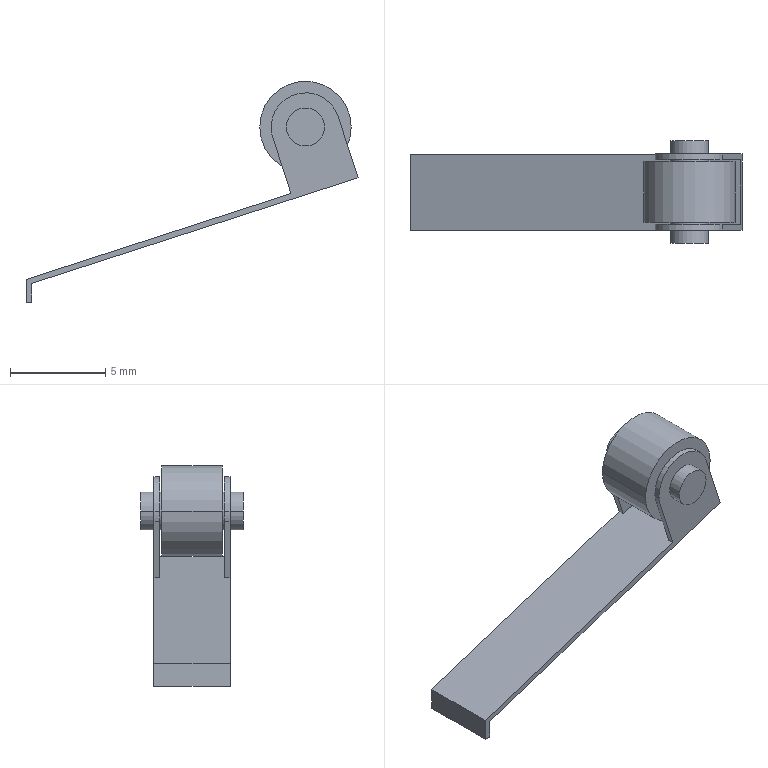Component | SolidWorks | SS_10GL2-1_SS_10GL2_ACTUATOR-1 | 1 solid | 30 faces | box 17.42 x 5.4 x 11.6 mm | volume 96 mm3 | plane 16 | cylinder 14 | commonest cylinder face diameters 2 x8 3.6 x4 4.8 x2
STEP:
#1=COLOUR_RGB('',0.7922,0.8196,0.9333);
#2=FILL_AREA_STYLE_COLOUR('',#1);
#3=FILL_AREA_STYLE('',(#2));
#4=SURFACE_STYLE_FILL_AREA(#3);
#5=SURFACE_SIDE_STYLE('',(#4));
#6=SURFACE_STYLE_USAGE(.BOTH.,#5);
#7=PRESENTATION_STYLE_ASSIGNMENT((#6));
#8=CARTESIAN_POINT('',(11.66,-32.095,0.3882));
#9=VERTEX_POINT('',#8);
#10=CARTESIAN_POINT('',(11.581,-32.095,0.3882));
#11=VERTEX_POINT('',#10);
#12=CARTESIAN_POINT('',(11.621,-32.095,0.3882));
#13=DIRECTION('',(0.,-1.,-0.));
#14=DIRECTION('',(1.,0.,0.));
#15=AXIS2_PLACEMENT_3D('',#12,#13,#14);
#16=CIRCLE('',#15,0.03937);
#17=EDGE_CURVE('',#9,#11,#16,.T.);
#18=ORIENTED_EDGE('',*,*,#17,.T.);
#19=CARTESIAN_POINT('',(11.581,-32.122,0.3882));
#20=VERTEX_POINT('',#19);
#21=CARTESIAN_POINT('',(11.581,-32.095,0.3882));
#22=DIRECTION('',(0.,-1.,-0.));
#23=VECTOR('',#22,39.37);
#24=LINE('',#21,#23);
#25=EDGE_CURVE('',#11,#20,#24,.T.);
#26=ORIENTED_EDGE('',*,*,#25,.T.);
#27=CARTESIAN_POINT('',(11.66,-32.122,0.3882));
#28=VERTEX_POINT('',#27);
#29=CARTESIAN_POINT('',(11.621,-32.122,0.3882));
#30=DIRECTION('',(0.,-1.,-0.));
#31=DIRECTION('',(1.,0.,0.));
#32=AXIS2_PLACEMENT_3D('',#29,#30,#31);
#33=CIRCLE('',#32,0.03937);
#34=EDGE_CURVE('',#28,#20,#33,.T.);
#35=ORIENTED_EDGE('',*,*,#34,.F.);
#36=CARTESIAN_POINT('',(11.66,-32.095,0.3882));
#37=DIRECTION('',(0.,-1.,-0.));
#38=VECTOR('',#37,39.37);
#39=LINE('',#36,#38);
#40=EDGE_CURVE('',#9,#28,#39,.T.);
#41=ORIENTED_EDGE('',*,*,#40,.F.);
#42=EDGE_LOOP('',(#18,#26,#35,#41));
#43=FACE_OUTER_BOUND('',#42,.T.);
#44=CARTESIAN_POINT('',(11.621,-32.095,0.3882));
#45=DIRECTION('',(0.,-1.,-0.));
#46=DIRECTION('',(1.,0.,0.));
#47=AXIS2_PLACEMENT_3D('',#44,#45,#46);
#48=CYLINDRICAL_SURFACE('',#47,0.03937);
#49=ADVANCED_FACE('',(#43),#48,.T.);
#50=CARTESIAN_POINT('',(11.553,-32.134,0.3664));
#51=VERTEX_POINT('',#50);
#52=CARTESIAN_POINT('',(11.55,-32.134,0.3882));
#53=VERTEX_POINT('',#52);
#54=CARTESIAN_POINT('',(11.621,-32.134,0.3882));
#55=DIRECTION('',(-0.,1.,0.));
#56=DIRECTION('',(-1.,0.,-0.));
#57=AXIS2_PLACEMENT_3D('',#54,#55,#56);
#58=CIRCLE('',#57,0.07087);
#59=EDGE_CURVE('',#51,#53,#58,.T.);
#60=ORIENTED_EDGE('',*,*,#59,.T.);
#61=CARTESIAN_POINT('',(11.55,-32.122,0.3882));
#62=VERTEX_POINT('',#61);
#63=CARTESIAN_POINT('',(11.55,-32.28,0.3882));
#64=DIRECTION('',(-0.,1.,0.));
#65=VECTOR('',#64,39.37);
#66=LINE('',#63,#65);
#67=EDGE_CURVE('',#53,#62,#66,.T.);
#68=ORIENTED_EDGE('',*,*,#67,.T.);
#69=CARTESIAN_POINT('',(11.553,-32.122,0.3664));
#70=VERTEX_POINT('',#69);
#71=CARTESIAN_POINT('',(11.621,-32.122,0.3882));
#72=DIRECTION('',(-0.,1.,0.));
#73=DIRECTION('',(-1.,0.,-0.));
#74=AXIS2_PLACEMENT_3D('',#71,#72,#73);
#75=CIRCLE('',#74,0.07087);
#76=EDGE_CURVE('',#70,#62,#75,.T.);
#77=ORIENTED_EDGE('',*,*,#76,.F.);
#78=CARTESIAN_POINT('',(11.553,-32.28,0.3664));
#79=DIRECTION('',(0.,-1.,-0.));
#80=VECTOR('',#79,39.37);
#81=LINE('',#78,#80);
#82=EDGE_CURVE('',#70,#51,#81,.T.);
#83=ORIENTED_EDGE('',*,*,#82,.T.);
#84=EDGE_LOOP('',(#60,#68,#77,#83));
#85=FACE_OUTER_BOUND('',#84,.T.);
#86=CARTESIAN_POINT('',(11.621,-32.28,0.3882));
#87=DIRECTION('',(-0.,1.,0.));
#88=DIRECTION('',(-1.,0.,-0.));
#89=AXIS2_PLACEMENT_3D('',#86,#87,#88);
#90=CYLINDRICAL_SURFACE('',#89,0.07087);
#91=ADVANCED_FACE('',(#85),#90,.T.);
#92=CARTESIAN_POINT('',(11.581,-32.307,0.3882));
#93=VERTEX_POINT('',#92);
#94=CARTESIAN_POINT('',(11.66,-32.307,0.3882));
#95=VERTEX_POINT('',#94);
#96=CARTESIAN_POINT('',(11.621,-32.307,0.3882));
#97=DIRECTION('',(-0.,1.,0.));
#98=DIRECTION('',(-1.,0.,-0.));
#99=AXIS2_PLACEMENT_3D('',#96,#97,#98);
#100=CIRCLE('',#99,0.03937);
#101=EDGE_CURVE('',#93,#95,#100,.T.);
#102=ORIENTED_EDGE('',*,*,#101,.T.);
#103=CARTESIAN_POINT('',(11.66,-32.28,0.3882));
#104=VERTEX_POINT('',#103);
#105=CARTESIAN_POINT('',(11.66,-32.307,0.3882));
#106=DIRECTION('',(-0.,1.,0.));
#107=VECTOR('',#106,39.37);
#108=LINE('',#105,#107);
#109=EDGE_CURVE('',#95,#104,#108,.T.);
#110=ORIENTED_EDGE('',*,*,#109,.T.);
#111=CARTESIAN_POINT('',(11.581,-32.28,0.3882));
#112=VERTEX_POINT('',#111);
#113=CARTESIAN_POINT('',(11.621,-32.28,0.3882));
#114=DIRECTION('',(0.,-1.,-0.));
#115=DIRECTION('',(-1.,0.,-0.));
#116=AXIS2_PLACEMENT_3D('',#113,#114,#115);
#117=CIRCLE('',#116,0.03937);
#118=EDGE_CURVE('',#104,#112,#117,.T.);
#119=ORIENTED_EDGE('',*,*,#118,.T.);
#120=CARTESIAN_POINT('',(11.581,-32.307,0.3882));
#121=DIRECTION('',(-0.,1.,0.));
#122=VECTOR('',#121,39.37);
#123=LINE('',#120,#122);
#124=EDGE_CURVE('',#93,#112,#123,.T.);
#125=ORIENTED_EDGE('',*,*,#124,.F.);
#126=EDGE_LOOP('',(#102,#110,#119,#125));
#127=FACE_OUTER_BOUND('',#126,.T.);
#128=CARTESIAN_POINT('',(11.621,-32.307,0.3882));
#129=DIRECTION('',(-0.,1.,0.));
#130=DIRECTION('',(-1.,0.,-0.));
#131=AXIS2_PLACEMENT_3D('',#128,#129,#130);
#132=CYLINDRICAL_SURFACE('',#131,0.03937);
#133=ADVANCED_FACE('',(#127),#132,.T.);
#134=CARTESIAN_POINT('',(11.553,-32.28,0.3664));
#135=VERTEX_POINT('',#134);
#136=CARTESIAN_POINT('',(11.55,-32.28,0.3882));
#137=VERTEX_POINT('',#136);
#138=CARTESIAN_POINT('',(11.621,-32.28,0.3882));
#139=DIRECTION('',(-0.,1.,0.));
#140=DIRECTION('',(-1.,0.,-0.));
#141=AXIS2_PLACEMENT_3D('',#138,#139,#140);
#142=CIRCLE('',#141,0.07087);
#143=EDGE_CURVE('',#135,#137,#142,.T.);
#144=ORIENTED_EDGE('',*,*,#143,.T.);
#145=CARTESIAN_POINT('',(11.55,-32.268,0.3882));
#146=VERTEX_POINT('',#145);
#147=CARTESIAN_POINT('',(11.55,-32.28,0.3882));
#148=DIRECTION('',(-0.,1.,0.));
#149=VECTOR('',#148,39.37);
#150=LINE('',#147,#149);
#151=EDGE_CURVE('',#137,#146,#150,.T.);
#152=ORIENTED_EDGE('',*,*,#151,.T.);
#153=CARTESIAN_POINT('',(11.553,-32.268,0.3664));
#154=VERTEX_POINT('',#153);
#155=CARTESIAN_POINT('',(11.621,-32.268,0.3882));
#156=DIRECTION('',(-0.,1.,0.));
#157=DIRECTION('',(-1.,0.,-0.));
#158=AXIS2_PLACEMENT_3D('',#155,#156,#157);
#159=CIRCLE('',#158,0.07087);
#160=EDGE_CURVE('',#154,#146,#159,.T.);
#161=ORIENTED_EDGE('',*,*,#160,.F.);
#162=CARTESIAN_POINT('',(11.553,-32.28,0.3664));
#163=DIRECTION('',(0.,-1.,-0.));
#164=VECTOR('',#163,39.37);
#165=LINE('',#162,#164);
#166=EDGE_CURVE('',#154,#135,#165,.T.);
#167=ORIENTED_EDGE('',*,*,#166,.T.);
#168=EDGE_LOOP('',(#144,#152,#161,#167));
#169=FACE_OUTER_BOUND('',#168,.T.);
#170=CARTESIAN_POINT('',(11.621,-32.28,0.3882));
#171=DIRECTION('',(-0.,1.,0.));
#172=DIRECTION('',(-1.,0.,-0.));
#173=AXIS2_PLACEMENT_3D('',#170,#171,#172);
#174=CYLINDRICAL_SURFACE('',#173,0.07087);
#175=ADVANCED_FACE('',(#169),#174,.T.);
#176=CARTESIAN_POINT('',(11.66,-32.268,0.3882));
#177=VERTEX_POINT('',#176);
#178=CARTESIAN_POINT('',(11.581,-32.268,0.3882));
#179=VERTEX_POINT('',#178);
#180=CARTESIAN_POINT('',(11.621,-32.268,0.3882));
#181=DIRECTION('',(0.,-1.,-0.));
#182=DIRECTION('',(-1.,0.,-0.));
#183=AXIS2_PLACEMENT_3D('',#180,#181,#182);
#184=CIRCLE('',#183,0.03937);
#185=EDGE_CURVE('',#177,#179,#184,.T.);
#186=ORIENTED_EDGE('',*,*,#185,.F.);
#187=CARTESIAN_POINT('',(11.66,-32.264,0.3882));
#188=VERTEX_POINT('',#187);
#189=CARTESIAN_POINT('',(11.66,-32.307,0.3882));
#190=DIRECTION('',(-0.,1.,0.));
#191=VECTOR('',#190,39.37);
#192=LINE('',#189,#191);
#193=EDGE_CURVE('',#177,#188,#192,.T.);
#194=ORIENTED_EDGE('',*,*,#193,.T.);
#195=CARTESIAN_POINT('',(11.581,-32.264,0.3882));
#196=VERTEX_POINT('',#195);
#197=CARTESIAN_POINT('',(11.621,-32.264,0.3882));
#198=DIRECTION('',(0.,-1.,-0.));
#199=DIRECTION('',(-1.,0.,-0.));
#200=AXIS2_PLACEMENT_3D('',#197,#198,#199);
#201=CIRCLE('',#200,0.03937);
#202=EDGE_CURVE('',#188,#196,#201,.T.);
#203=ORIENTED_EDGE('',*,*,#202,.T.);
#204=CARTESIAN_POINT('',(11.581,-32.307,0.3882));
#205=DIRECTION('',(-0.,1.,0.));
#206=VECTOR('',#205,39.37);
#207=LINE('',#204,#206);
#208=EDGE_CURVE('',#179,#196,#207,.T.);
#209=ORIENTED_EDGE('',*,*,#208,.F.);
#210=EDGE_LOOP('',(#186,#194,#203,#209));
#211=FACE_OUTER_BOUND('',#210,.T.);
#212=CARTESIAN_POINT('',(11.621,-32.307,0.3882));
#213=DIRECTION('',(-0.,1.,0.));
#214=DIRECTION('',(-1.,0.,-0.));
#215=AXIS2_PLACEMENT_3D('',#212,#213,#214);
#216=CYLINDRICAL_SURFACE('',#215,0.03937);
#217=ADVANCED_FACE('',(#211),#216,.T.);
#218=CARTESIAN_POINT('',(11.66,-32.134,0.3882));
#219=VERTEX_POINT('',#218);
#220=CARTESIAN_POINT('',(11.581,-32.134,0.3882));
#221=VERTEX_POINT('',#220);
#222=CARTESIAN_POINT('',(11.621,-32.134,0.3882));
#223=DIRECTION('',(0.,-1.,-0.));
#224=DIRECTION('',(1.,0.,0.));
#225=AXIS2_PLACEMENT_3D('',#222,#223,#224);
#226=CIRCLE('',#225,0.03937);
#227=EDGE_CURVE('',#219,#221,#226,.T.);
#228=ORIENTED_EDGE('',*,*,#227,.T.);
#229=CARTESIAN_POINT('',(11.581,-32.138,0.3882));
#230=VERTEX_POINT('',#229);
#231=CARTESIAN_POINT('',(11.581,-32.095,0.3882));
#232=DIRECTION('',(0.,-1.,-0.));
#233=VECTOR('',#232,39.37);
#234=LINE('',#231,#233);
#235=EDGE_CURVE('',#221,#230,#234,.T.);
#236=ORIENTED_EDGE('',*,*,#235,.T.);
#237=CARTESIAN_POINT('',(11.66,-32.138,0.3882));
#238=VERTEX_POINT('',#237);
#239=CARTESIAN_POINT('',(11.621,-32.138,0.3882));
#240=DIRECTION('',(-0.,1.,0.));
#241=DIRECTION('',(1.,0.,0.));
#242=AXIS2_PLACEMENT_3D('',#239,#240,#241);
#243=CIRCLE('',#242,0.03937);
#244=EDGE_CURVE('',#230,#238,#243,.T.);
#245=ORIENTED_EDGE('',*,*,#244,.T.);
#246=CARTESIAN_POINT('',(11.66,-32.095,0.3882));
#247=DIRECTION('',(0.,-1.,-0.));
#248=VECTOR('',#247,39.37);
#249=LINE('',#246,#248);
#250=EDGE_CURVE('',#219,#238,#249,.T.);
#251=ORIENTED_EDGE('',*,*,#250,.F.);
#252=EDGE_LOOP('',(#228,#236,#245,#251));
#253=FACE_OUTER_BOUND('',#252,.T.);
#254=CARTESIAN_POINT('',(11.621,-32.095,0.3882));
#255=DIRECTION('',(0.,-1.,-0.));
#256=DIRECTION('',(1.,0.,0.));
#257=AXIS2_PLACEMENT_3D('',#254,#255,#256);
#258=CYLINDRICAL_SURFACE('',#257,0.03937);
#259=ADVANCED_FACE('',(#253),#258,.T.);
#260=CARTESIAN_POINT('',(11.526,-32.138,0.3882));
#261=VERTEX_POINT('',#260);
#262=CARTESIAN_POINT('',(11.715,-32.138,0.3882));
#263=VERTEX_POINT('',#262);
#264=CARTESIAN_POINT('',(11.621,-32.138,0.3882));
#265=DIRECTION('',(-0.,1.,0.));
#266=DIRECTION('',(1.,0.,0.));
#267=AXIS2_PLACEMENT_3D('',#264,#265,#266);
#268=CIRCLE('',#267,0.09449);
#269=EDGE_CURVE('',#261,#263,#268,.T.);
#270=ORIENTED_EDGE('',*,*,#269,.F.);
#271=CARTESIAN_POINT('',(11.526,-32.264,0.3882));
#272=VERTEX_POINT('',#271);
#273=CARTESIAN_POINT('',(11.526,-32.138,0.3882));
#274=DIRECTION('',(0.,-1.,-0.));
#275=VECTOR('',#274,39.37);
#276=LINE('',#273,#275);
#277=EDGE_CURVE('',#261,#272,#276,.T.);
#278=ORIENTED_EDGE('',*,*,#277,.T.);
#279=CARTESIAN_POINT('',(11.715,-32.264,0.3882));
#280=VERTEX_POINT('',#279);
#281=CARTESIAN_POINT('',(11.621,-32.264,0.3882));
#282=DIRECTION('',(-0.,1.,0.));
#283=DIRECTION('',(1.,0.,0.));
#284=AXIS2_PLACEMENT_3D('',#281,#282,#283);
#285=CIRCLE('',#284,0.09449);
#286=EDGE_CURVE('',#272,#280,#285,.T.);
#287=ORIENTED_EDGE('',*,*,#286,.T.);
#288=CARTESIAN_POINT('',(11.715,-32.138,0.3882));
#289=DIRECTION('',(0.,-1.,-0.));
#290=VECTOR('',#289,39.37);
#291=LINE('',#288,#290);
#292=EDGE_CURVE('',#263,#280,#291,.T.);
#293=ORIENTED_EDGE('',*,*,#292,.F.);
#294=EDGE_LOOP('',(#270,#278,#287,#293));
#295=FACE_OUTER_BOUND('',#294,.T.);
#296=CARTESIAN_POINT('',(11.621,-32.138,0.3882));
#297=DIRECTION('',(0.,-1.,-0.));
#298=DIRECTION('',(1.,0.,0.));
#299=AXIS2_PLACEMENT_3D('',#296,#297,#298);
#300=CYLINDRICAL_SURFACE('',#299,0.09449);
#301=ADVANCED_FACE('',(#295),#300,.T.);
#302=CARTESIAN_POINT('',(11.729,-32.28,0.2829));
#303=VERTEX_POINT('',#302);
#304=CARTESIAN_POINT('',(11.729,-32.122,0.2829));
#305=VERTEX_POINT('',#304);
#306=CARTESIAN_POINT('',(11.729,-32.28,0.2829));
#307=DIRECTION('',(-0.,1.,0.));
#308=VECTOR('',#307,39.37);
#309=LINE('',#306,#308);
#310=EDGE_CURVE('',#303,#305,#309,.T.);
#311=ORIENTED_EDGE('',*,*,#310,.F.);
#312=CARTESIAN_POINT('',(11.055,-32.28,0.06494));
#313=VERTEX_POINT('',#312);
#314=CARTESIAN_POINT('',(11.055,-32.28,0.06494));
#315=DIRECTION('',(0.9515,0.,0.3077));
#316=VECTOR('',#315,39.37);
#317=LINE('',#314,#316);
#318=EDGE_CURVE('',#313,#303,#317,.T.);
#319=ORIENTED_EDGE('',*,*,#318,.F.);
#320=CARTESIAN_POINT('',(11.055,-32.122,0.06494));
#321=VERTEX_POINT('',#320);
#322=CARTESIAN_POINT('',(11.055,-32.28,0.06494));
#323=DIRECTION('',(0.,-1.,-0.));
#324=VECTOR('',#323,39.37);
#325=LINE('',#322,#324);
#326=EDGE_CURVE('',#321,#313,#325,.T.);
#327=ORIENTED_EDGE('',*,*,#326,.F.);
#328=CARTESIAN_POINT('',(11.055,-32.122,0.06494));
#329=DIRECTION('',(-0.9515,-0.,-0.3077));
#330=VECTOR('',#329,39.37);
#331=LINE('',#328,#330);
#332=EDGE_CURVE('',#305,#321,#331,.T.);
#333=ORIENTED_EDGE('',*,*,#332,.F.);
#334=EDGE_LOOP('',(#311,#319,#327,#333));
#335=FACE_OUTER_BOUND('',#334,.T.);
#336=CARTESIAN_POINT('',(11.055,-32.28,0.06494));
#337=DIRECTION('',(-0.3077,-0.,0.9515));
#338=DIRECTION('',(-0.9515,-0.,-0.3077));
#339=AXIS2_PLACEMENT_3D('',#336,#337,#338);
#340=PLANE('',#339);
#341=ADVANCED_FACE('',(#335),#340,.F.);
#342=ORIENTED_EDGE('',*,*,#34,.T.);
#343=CARTESIAN_POINT('',(11.621,-32.122,0.3882));
#344=DIRECTION('',(0.,-1.,-0.));
#345=DIRECTION('',(1.,0.,0.));
#346=AXIS2_PLACEMENT_3D('',#343,#344,#345);
#347=CIRCLE('',#346,0.03937);
#348=EDGE_CURVE('',#20,#28,#347,.T.);
#349=ORIENTED_EDGE('',*,*,#348,.T.);
#350=EDGE_LOOP('',(#342,#349));
#351=FACE_BOUND('',#350,.T.);
#352=CARTESIAN_POINT('',(11.688,-32.122,0.41));
#353=VERTEX_POINT('',#352);
#354=CARTESIAN_POINT('',(11.688,-32.122,0.41));
#355=DIRECTION('',(0.3077,0.,-0.9515));
#356=VECTOR('',#355,39.37);
#357=LINE('',#354,#356);
#358=EDGE_CURVE('',#353,#305,#357,.T.);
#359=ORIENTED_EDGE('',*,*,#358,.T.);
#360=ORIENTED_EDGE('',*,*,#332,.T.);
#361=CARTESIAN_POINT('',(11.055,-32.122,0.02597));
#362=VERTEX_POINT('',#361);
#363=CARTESIAN_POINT('',(11.055,-32.122,0.3882));
#364=DIRECTION('',(0.,0.,-1.));
#365=VECTOR('',#364,39.37);
#366=LINE('',#363,#365);
#367=EDGE_CURVE('',#321,#362,#366,.T.);
#368=ORIENTED_EDGE('',*,*,#367,.T.);
#369=CARTESIAN_POINT('',(11.043,-32.122,0.02597));
#370=VERTEX_POINT('',#369);
#371=CARTESIAN_POINT('',(11.055,-32.122,0.02597));
#372=DIRECTION('',(-1.,-0.,-0.));
#373=VECTOR('',#372,39.37);
#374=LINE('',#371,#373);
#375=EDGE_CURVE('',#362,#370,#374,.T.);
#376=ORIENTED_EDGE('',*,*,#375,.T.);
#377=CARTESIAN_POINT('',(11.043,-32.122,0.07354));
#378=VERTEX_POINT('',#377);
#379=CARTESIAN_POINT('',(11.043,-32.122,0.07354));
#380=DIRECTION('',(-0.,-0.,1.));
#381=VECTOR('',#380,39.37);
#382=LINE('',#379,#381);
#383=EDGE_CURVE('',#370,#378,#382,.T.);
#384=ORIENTED_EDGE('',*,*,#383,.T.);
#385=CARTESIAN_POINT('',(11.591,-32.122,0.2506));
#386=VERTEX_POINT('',#385);
#387=CARTESIAN_POINT('',(11.043,-32.122,0.07354));
#388=DIRECTION('',(0.9515,0.,0.3077));
#389=VECTOR('',#388,39.37);
#390=LINE('',#387,#389);
#391=EDGE_CURVE('',#378,#386,#390,.T.);
#392=ORIENTED_EDGE('',*,*,#391,.T.);
#393=CARTESIAN_POINT('',(11.591,-32.122,0.2506));
#394=DIRECTION('',(-0.3077,-0.,0.9515));
#395=VECTOR('',#394,39.37);
#396=LINE('',#393,#395);
#397=EDGE_CURVE('',#386,#70,#396,.T.);
#398=ORIENTED_EDGE('',*,*,#397,.T.);
#399=ORIENTED_EDGE('',*,*,#76,.T.);
#400=CARTESIAN_POINT('',(11.621,-32.122,0.3882));
#401=DIRECTION('',(-0.,1.,0.));
#402=DIRECTION('',(-1.,0.,-0.));
#403=AXIS2_PLACEMENT_3D('',#400,#401,#402);
#404=CIRCLE('',#403,0.07087);
#405=EDGE_CURVE('',#62,#353,#404,.T.);
#406=ORIENTED_EDGE('',*,*,#405,.T.);
#407=EDGE_LOOP('',(#359,#360,#368,#376,#384,#392,#398,#399,#406));
#408=FACE_OUTER_BOUND('',#407,.T.);
#409=CARTESIAN_POINT('',(11.621,-32.122,0.3882));
#410=DIRECTION('',(-0.,1.,0.));
#411=DIRECTION('',(-1.,-0.,-0.));
#412=AXIS2_PLACEMENT_3D('',#409,#410,#411);
#413=PLANE('',#412);
#414=ADVANCED_FACE('',(#351,#408),#413,.T.);
#415=CARTESIAN_POINT('',(11.688,-32.28,0.41));
#416=VERTEX_POINT('',#415);
#417=CARTESIAN_POINT('',(11.688,-32.268,0.41));
#418=VERTEX_POINT('',#417);
#419=CARTESIAN_POINT('',(11.688,-32.28,0.41));
#420=DIRECTION('',(-0.,1.,0.));
#421=VECTOR('',#420,39.37);
#422=LINE('',#419,#421);
#423=EDGE_CURVE('',#416,#418,#422,.T.);
#424=ORIENTED_EDGE('',*,*,#423,.F.);
#425=CARTESIAN_POINT('',(11.688,-32.28,0.41));
#426=DIRECTION('',(-0.3077,-0.,0.9515));
#427=VECTOR('',#426,39.37);
#428=LINE('',#425,#427);
#429=EDGE_CURVE('',#303,#416,#428,.T.);
#430=ORIENTED_EDGE('',*,*,#429,.F.);
#431=ORIENTED_EDGE('',*,*,#310,.T.);
#432=ORIENTED_EDGE('',*,*,#358,.F.);
#433=CARTESIAN_POINT('',(11.688,-32.134,0.41));
#434=VERTEX_POINT('',#433);
#435=CARTESIAN_POINT('',(11.688,-32.28,0.41));
#436=DIRECTION('',(-0.,1.,0.));
#437=VECTOR('',#436,39.37);
#438=LINE('',#435,#437);
#439=EDGE_CURVE('',#434,#353,#438,.T.);
#440=ORIENTED_EDGE('',*,*,#439,.F.);
#441=CARTESIAN_POINT('',(11.726,-32.134,0.2942));
#442=VERTEX_POINT('',#441);
#443=CARTESIAN_POINT('',(11.688,-32.134,0.41));
#444=DIRECTION('',(-0.3077,-0.,0.9515));
#445=VECTOR('',#444,39.37);
#446=LINE('',#443,#445);
#447=EDGE_CURVE('',#442,#434,#446,.T.);
#448=ORIENTED_EDGE('',*,*,#447,.F.);
#449=CARTESIAN_POINT('',(11.726,-32.268,0.2942));
#450=VERTEX_POINT('',#449);
#451=CARTESIAN_POINT('',(11.726,-32.28,0.2942));
#452=DIRECTION('',(-0.,1.,0.));
#453=VECTOR('',#452,39.37);
#454=LINE('',#451,#453);
#455=EDGE_CURVE('',#450,#442,#454,.T.);
#456=ORIENTED_EDGE('',*,*,#455,.F.);
#457=CARTESIAN_POINT('',(11.688,-32.268,0.41));
#458=DIRECTION('',(0.3077,0.,-0.9515));
#459=VECTOR('',#458,39.37);
#460=LINE('',#457,#459);
#461=EDGE_CURVE('',#418,#450,#460,.T.);
#462=ORIENTED_EDGE('',*,*,#461,.F.);
#463=EDGE_LOOP('',(#424,#430,#431,#432,#440,#448,#456,#462));
#464=FACE_OUTER_BOUND('',#463,.T.);
#465=CARTESIAN_POINT('',(11.688,-32.28,0.41));
#466=DIRECTION('',(-0.9515,-0.,-0.3077));
#467=DIRECTION('',(0.3077,0.,-0.9515));
#468=AXIS2_PLACEMENT_3D('',#465,#466,#467);
#469=PLANE('',#468);
#470=ADVANCED_FACE('',(#464),#469,.F.);
#471=CARTESIAN_POINT('',(11.621,-32.28,0.3882));
#472=DIRECTION('',(0.,-1.,-0.));
#473=DIRECTION('',(-1.,0.,-0.));
#474=AXIS2_PLACEMENT_3D('',#471,#472,#473);
#475=CIRCLE('',#474,0.03937);
#476=EDGE_CURVE('',#112,#104,#475,.T.);
#477=ORIENTED_EDGE('',*,*,#476,.F.);
#478=ORIENTED_EDGE('',*,*,#118,.F.);
#479=EDGE_LOOP('',(#477,#478));
#480=FACE_BOUND('',#479,.T.);
#481=ORIENTED_EDGE('',*,*,#318,.T.);
#482=ORIENTED_EDGE('',*,*,#429,.T.);
#483=CARTESIAN_POINT('',(11.621,-32.28,0.3882));
#484=DIRECTION('',(-0.,1.,0.));
#485=DIRECTION('',(-1.,0.,-0.));
#486=AXIS2_PLACEMENT_3D('',#483,#484,#485);
#487=CIRCLE('',#486,0.07087);
#488=EDGE_CURVE('',#137,#416,#487,.T.);
#489=ORIENTED_EDGE('',*,*,#488,.F.);
#490=ORIENTED_EDGE('',*,*,#143,.F.);
#491=CARTESIAN_POINT('',(11.591,-32.28,0.2506));
#492=VERTEX_POINT('',#491);
#493=CARTESIAN_POINT('',(11.591,-32.28,0.2506));
#494=DIRECTION('',(-0.3077,-0.,0.9515));
#495=VECTOR('',#494,39.37);
#496=LINE('',#493,#495);
#497=EDGE_CURVE('',#492,#135,#496,.T.);
#498=ORIENTED_EDGE('',*,*,#497,.F.);
#499=CARTESIAN_POINT('',(11.043,-32.28,0.07354));
#500=VERTEX_POINT('',#499);
#501=CARTESIAN_POINT('',(11.043,-32.28,0.07354));
#502=DIRECTION('',(0.9515,0.,0.3077));
#503=VECTOR('',#502,39.37);
#504=LINE('',#501,#503);
#505=EDGE_CURVE('',#500,#492,#504,.T.);
#506=ORIENTED_EDGE('',*,*,#505,.F.);
#507=CARTESIAN_POINT('',(11.043,-32.28,0.02597));
#508=VERTEX_POINT('',#507);
#509=CARTESIAN_POINT('',(11.043,-32.28,0.07354));
#510=DIRECTION('',(0.,0.,-1.));
#511=VECTOR('',#510,39.37);
#512=LINE('',#509,#511);
#513=EDGE_CURVE('',#500,#508,#512,.T.);
#514=ORIENTED_EDGE('',*,*,#513,.T.);
#515=CARTESIAN_POINT('',(11.055,-32.28,0.02597));
#516=VERTEX_POINT('',#515);
#517=CARTESIAN_POINT('',(11.055,-32.28,0.02597));
#518=DIRECTION('',(1.,0.,0.));
#519=VECTOR('',#518,39.37);
#520=LINE('',#517,#519);
#521=EDGE_CURVE('',#508,#516,#520,.T.);
#522=ORIENTED_EDGE('',*,*,#521,.T.);
#523=CARTESIAN_POINT('',(11.055,-32.28,0.3882));
#524=DIRECTION('',(0.,0.,-1.));
#525=VECTOR('',#524,39.37);
#526=LINE('',#523,#525);
#527=EDGE_CURVE('',#313,#516,#526,.T.);
#528=ORIENTED_EDGE('',*,*,#527,.F.);
#529=EDGE_LOOP('',(#481,#482,#489,#490,#498,#506,#514,#522,#528));
#530=FACE_OUTER_BOUND('',#529,.T.);
#531=CARTESIAN_POINT('',(11.621,-32.28,0.3882));
#532=DIRECTION('',(-0.,1.,0.));
#533=DIRECTION('',(-1.,-0.,-0.));
#534=AXIS2_PLACEMENT_3D('',#531,#532,#533);
#535=PLANE('',#534);
#536=ADVANCED_FACE('',(#480,#530),#535,.F.);
#537=ORIENTED_EDGE('',*,*,#326,.T.);
#538=ORIENTED_EDGE('',*,*,#527,.T.);
#539=CARTESIAN_POINT('',(11.055,-32.28,0.02597));
#540=DIRECTION('',(0.,-1.,-0.));
#541=VECTOR('',#540,39.37);
#542=LINE('',#539,#541);
#543=EDGE_CURVE('',#362,#516,#542,.T.);
#544=ORIENTED_EDGE('',*,*,#543,.F.);
#545=ORIENTED_EDGE('',*,*,#367,.F.);
#546=EDGE_LOOP('',(#537,#538,#544,#545));
#547=FACE_OUTER_BOUND('',#546,.T.);
#548=CARTESIAN_POINT('',(11.055,-32.28,0.02597));
#549=DIRECTION('',(-1.,-0.,-0.));
#550=DIRECTION('',(0.,-1.,-0.));
#551=AXIS2_PLACEMENT_3D('',#548,#549,#550);
#552=PLANE('',#551);
#553=ADVANCED_FACE('',(#547),#552,.F.);
#554=ORIENTED_EDGE('',*,*,#25,.F.);
#555=CARTESIAN_POINT('',(11.621,-32.095,0.3882));
#556=DIRECTION('',(0.,-1.,-0.));
#557=DIRECTION('',(1.,0.,0.));
#558=AXIS2_PLACEMENT_3D('',#555,#556,#557);
#559=CIRCLE('',#558,0.03937);
#560=EDGE_CURVE('',#11,#9,#559,.T.);
#561=ORIENTED_EDGE('',*,*,#560,.T.);
#562=ORIENTED_EDGE('',*,*,#40,.T.);
#563=ORIENTED_EDGE('',*,*,#348,.F.);
#564=EDGE_LOOP('',(#554,#561,#562,#563));
#565=FACE_OUTER_BOUND('',#564,.T.);
#566=CARTESIAN_POINT('',(11.621,-32.095,0.3882));
#567=DIRECTION('',(0.,-1.,-0.));
#568=DIRECTION('',(1.,0.,0.));
#569=AXIS2_PLACEMENT_3D('',#566,#567,#568);
#570=CYLINDRICAL_SURFACE('',#569,0.03937);
#571=ADVANCED_FACE('',(#565),#570,.T.);
#572=ORIENTED_EDGE('',*,*,#67,.F.);
#573=CARTESIAN_POINT('',(11.621,-32.134,0.3882));
#574=DIRECTION('',(-0.,1.,0.));
#575=DIRECTION('',(-1.,0.,-0.));
#576=AXIS2_PLACEMENT_3D('',#573,#574,#575);
#577=CIRCLE('',#576,0.07087);
#578=EDGE_CURVE('',#53,#434,#577,.T.);
#579=ORIENTED_EDGE('',*,*,#578,.T.);
#580=ORIENTED_EDGE('',*,*,#439,.T.);
#581=ORIENTED_EDGE('',*,*,#405,.F.);
#582=EDGE_LOOP('',(#572,#579,#580,#581));
#583=FACE_OUTER_BOUND('',#582,.T.);
#584=CARTESIAN_POINT('',(11.621,-32.28,0.3882));
#585=DIRECTION('',(-0.,1.,0.));
#586=DIRECTION('',(-1.,0.,-0.));
#587=AXIS2_PLACEMENT_3D('',#584,#585,#586);
#588=CYLINDRICAL_SURFACE('',#587,0.07087);
#589=ADVANCED_FACE('',(#583),#588,.T.);
#590=CARTESIAN_POINT('',(11.591,-32.134,0.2506));
#591=VERTEX_POINT('',#590);
#592=CARTESIAN_POINT('',(11.591,-32.134,0.2506));
#593=DIRECTION('',(0.3077,0.,-0.9515));
#594=VECTOR('',#593,39.37);
#595=LINE('',#592,#594);
#596=EDGE_CURVE('',#51,#591,#595,.T.);
#597=ORIENTED_EDGE('',*,*,#596,.F.);
#598=ORIENTED_EDGE('',*,*,#82,.F.);
#599=ORIENTED_EDGE('',*,*,#397,.F.);
#600=CARTESIAN_POINT('',(11.591,-32.28,0.2506));
#601=DIRECTION('',(-0.,1.,0.));
#602=VECTOR('',#601,39.37);
#603=LINE('',#600,#602);
#604=EDGE_CURVE('',#591,#386,#603,.T.);
#605=ORIENTED_EDGE('',*,*,#604,.F.);
#606=EDGE_LOOP('',(#597,#598,#599,#605));
#607=FACE_OUTER_BOUND('',#606,.T.);
#608=CARTESIAN_POINT('',(11.591,-32.28,0.2506));
#609=DIRECTION('',(0.9515,0.,0.3077));
#610=DIRECTION('',(-0.3077,-0.,0.9515));
#611=AXIS2_PLACEMENT_3D('',#608,#609,#610);
#612=PLANE('',#611);
#613=ADVANCED_FACE('',(#607),#612,.F.);
#614=CARTESIAN_POINT('',(11.043,-32.28,0.07354));
#615=DIRECTION('',(-0.,1.,0.));
#616=VECTOR('',#615,39.37);
#617=LINE('',#614,#616);
#618=EDGE_CURVE('',#500,#378,#617,.T.);
#619=ORIENTED_EDGE('',*,*,#618,.F.);
#620=ORIENTED_EDGE('',*,*,#505,.T.);
#621=CARTESIAN_POINT('',(11.591,-32.268,0.2506));
#622=VERTEX_POINT('',#621);
#623=CARTESIAN_POINT('',(11.591,-32.28,0.2506));
#624=DIRECTION('',(0.,-1.,-0.));
#625=VECTOR('',#624,39.37);
#626=LINE('',#623,#625);
#627=EDGE_CURVE('',#622,#492,#626,.T.);
#628=ORIENTED_EDGE('',*,*,#627,.F.);
#629=CARTESIAN_POINT('',(11.591,-32.268,0.2506));
#630=DIRECTION('',(-0.9515,-0.,-0.3077));
#631=VECTOR('',#630,39.37);
#632=LINE('',#629,#631);
#633=EDGE_CURVE('',#450,#622,#632,.T.);
#634=ORIENTED_EDGE('',*,*,#633,.F.);
#635=ORIENTED_EDGE('',*,*,#455,.T.);
#636=CARTESIAN_POINT('',(11.591,-32.134,0.2506));
#637=DIRECTION('',(0.9515,0.,0.3077));
#638=VECTOR('',#637,39.37);
#639=LINE('',#636,#638);
#640=EDGE_CURVE('',#591,#442,#639,.T.);
#641=ORIENTED_EDGE('',*,*,#640,.F.);
#642=ORIENTED_EDGE('',*,*,#604,.T.);
#643=ORIENTED_EDGE('',*,*,#391,.F.);
#644=EDGE_LOOP('',(#619,#620,#628,#634,#635,#641,#642,#643));
#645=FACE_OUTER_BOUND('',#644,.T.);
#646=CARTESIAN_POINT('',(11.591,-32.28,0.2506));
#647=DIRECTION('',(0.3077,0.,-0.9515));
#648=DIRECTION('',(0.9515,0.,0.3077));
#649=AXIS2_PLACEMENT_3D('',#646,#647,#648);
#650=PLANE('',#649);
#651=ADVANCED_FACE('',(#645),#650,.F.);
#652=CARTESIAN_POINT('',(11.621,-32.268,0.3882));
#653=DIRECTION('',(0.,-1.,-0.));
#654=DIRECTION('',(-1.,0.,-0.));
#655=AXIS2_PLACEMENT_3D('',#652,#653,#654);
#656=CIRCLE('',#655,0.03937);
#657=EDGE_CURVE('',#179,#177,#656,.T.);
#658=ORIENTED_EDGE('',*,*,#657,.T.);
#659=ORIENTED_EDGE('',*,*,#185,.T.);
#660=EDGE_LOOP('',(#658,#659));
#661=FACE_BOUND('',#660,.T.);
#662=ORIENTED_EDGE('',*,*,#160,.T.);
#663=CARTESIAN_POINT('',(11.621,-32.268,0.3882));
#664=DIRECTION('',(-0.,1.,0.));
#665=DIRECTION('',(-1.,0.,-0.));
#666=AXIS2_PLACEMENT_3D('',#663,#664,#665);
#667=CIRCLE('',#666,0.07087);
#668=EDGE_CURVE('',#146,#418,#667,.T.);
#669=ORIENTED_EDGE('',*,*,#668,.T.);
#670=ORIENTED_EDGE('',*,*,#461,.T.);
#671=ORIENTED_EDGE('',*,*,#633,.T.);
#672=CARTESIAN_POINT('',(11.591,-32.268,0.2506));
#673=DIRECTION('',(-0.3077,-0.,0.9515));
#674=VECTOR('',#673,39.37);
#675=LINE('',#672,#674);
#676=EDGE_CURVE('',#622,#154,#675,.T.);
#677=ORIENTED_EDGE('',*,*,#676,.T.);
#678=EDGE_LOOP('',(#662,#669,#670,#671,#677));
#679=FACE_OUTER_BOUND('',#678,.T.);
#680=CARTESIAN_POINT('',(11.621,-32.268,0.3882));
#681=DIRECTION('',(-0.,1.,0.));
#682=DIRECTION('',(-1.,-0.,-0.));
#683=AXIS2_PLACEMENT_3D('',#680,#681,#682);
#684=PLANE('',#683);
#685=ADVANCED_FACE('',(#661,#679),#684,.T.);
#686=ORIENTED_EDGE('',*,*,#227,.F.);
#687=CARTESIAN_POINT('',(11.621,-32.134,0.3882));
#688=DIRECTION('',(0.,-1.,-0.));
#689=DIRECTION('',(1.,0.,0.));
#690=AXIS2_PLACEMENT_3D('',#687,#688,#689);
#691=CIRCLE('',#690,0.03937);
#692=EDGE_CURVE('',#221,#219,#691,.T.);
#693=ORIENTED_EDGE('',*,*,#692,.F.);
#694=EDGE_LOOP('',(#686,#693));
#695=FACE_BOUND('',#694,.T.);
#696=ORIENTED_EDGE('',*,*,#640,.T.);
#697=ORIENTED_EDGE('',*,*,#447,.T.);
#698=ORIENTED_EDGE('',*,*,#578,.F.);
#699=ORIENTED_EDGE('',*,*,#59,.F.);
#700=ORIENTED_EDGE('',*,*,#596,.T.);
#701=EDGE_LOOP('',(#696,#697,#698,#699,#700));
#702=FACE_OUTER_BOUND('',#701,.T.);
#703=CARTESIAN_POINT('',(11.621,-32.134,0.3882));
#704=DIRECTION('',(-0.,1.,0.));
#705=DIRECTION('',(-1.,-0.,-0.));
#706=AXIS2_PLACEMENT_3D('',#703,#704,#705);
#707=PLANE('',#706);
#708=ADVANCED_FACE('',(#695,#702),#707,.F.);
#709=ORIENTED_EDGE('',*,*,#109,.F.);
#710=CARTESIAN_POINT('',(11.621,-32.307,0.3882));
#711=DIRECTION('',(-0.,1.,0.));
#712=DIRECTION('',(-1.,0.,-0.));
#713=AXIS2_PLACEMENT_3D('',#710,#711,#712);
#714=CIRCLE('',#713,0.03937);
#715=EDGE_CURVE('',#95,#93,#714,.T.);
#716=ORIENTED_EDGE('',*,*,#715,.T.);
#717=ORIENTED_EDGE('',*,*,#124,.T.);
#718=ORIENTED_EDGE('',*,*,#476,.T.);
#719=EDGE_LOOP('',(#709,#716,#717,#718));
#720=FACE_OUTER_BOUND('',#719,.T.);
#721=CARTESIAN_POINT('',(11.621,-32.307,0.3882));
#722=DIRECTION('',(-0.,1.,0.));
#723=DIRECTION('',(-1.,0.,-0.));
#724=AXIS2_PLACEMENT_3D('',#721,#722,#723);
#725=CYLINDRICAL_SURFACE('',#724,0.03937);
#726=ADVANCED_FACE('',(#720),#725,.T.);
#727=ORIENTED_EDGE('',*,*,#151,.F.);
#728=ORIENTED_EDGE('',*,*,#488,.T.);
#729=ORIENTED_EDGE('',*,*,#423,.T.);
#730=ORIENTED_EDGE('',*,*,#668,.F.);
#731=EDGE_LOOP('',(#727,#728,#729,#730));
#732=FACE_OUTER_BOUND('',#731,.T.);
#733=CARTESIAN_POINT('',(11.621,-32.28,0.3882));
#734=DIRECTION('',(-0.,1.,0.));
#735=DIRECTION('',(-1.,0.,-0.));
#736=AXIS2_PLACEMENT_3D('',#733,#734,#735);
#737=CYLINDRICAL_SURFACE('',#736,0.07087);
#738=ADVANCED_FACE('',(#732),#737,.T.);
#739=ORIENTED_EDGE('',*,*,#627,.T.);
#740=ORIENTED_EDGE('',*,*,#497,.T.);
#741=ORIENTED_EDGE('',*,*,#166,.F.);
#742=ORIENTED_EDGE('',*,*,#676,.F.);
#743=EDGE_LOOP('',(#739,#740,#741,#742));
#744=FACE_OUTER_BOUND('',#743,.T.);
#745=CARTESIAN_POINT('',(11.591,-32.28,0.2506));
#746=DIRECTION('',(0.9515,0.,0.3077));
#747=DIRECTION('',(-0.3077,-0.,0.9515));
#748=AXIS2_PLACEMENT_3D('',#745,#746,#747);
#749=PLANE('',#748);
#750=ADVANCED_FACE('',(#744),#749,.F.);
#751=ORIENTED_EDGE('',*,*,#543,.T.);
#752=ORIENTED_EDGE('',*,*,#521,.F.);
#753=CARTESIAN_POINT('',(11.043,-32.28,0.02597));
#754=DIRECTION('',(0.,-1.,-0.));
#755=VECTOR('',#754,39.37);
#756=LINE('',#753,#755);
#757=EDGE_CURVE('',#370,#508,#756,.T.);
#758=ORIENTED_EDGE('',*,*,#757,.F.);
#759=ORIENTED_EDGE('',*,*,#375,.F.);
#760=EDGE_LOOP('',(#751,#752,#758,#759));
#761=FACE_OUTER_BOUND('',#760,.T.);
#762=CARTESIAN_POINT('',(11.055,-32.28,0.02597));
#763=DIRECTION('',(-0.,-0.,1.));
#764=DIRECTION('',(0.,-1.,-0.));
#765=AXIS2_PLACEMENT_3D('',#762,#763,#764);
#766=PLANE('',#765);
#767=ADVANCED_FACE('',(#761),#766,.F.);
#768=ORIENTED_EDGE('',*,*,#17,.F.);
#769=ORIENTED_EDGE('',*,*,#560,.F.);
#770=EDGE_LOOP('',(#768,#769));
#771=FACE_OUTER_BOUND('',#770,.T.);
#772=CARTESIAN_POINT('',(11.621,-32.095,0.3882));
#773=DIRECTION('',(-0.,1.,0.));
#774=DIRECTION('',(-1.,-0.,-0.));
#775=AXIS2_PLACEMENT_3D('',#772,#773,#774);
#776=PLANE('',#775);
#777=ADVANCED_FACE('',(#771),#776,.T.);
#778=ORIENTED_EDGE('',*,*,#757,.T.);
#779=ORIENTED_EDGE('',*,*,#513,.F.);
#780=ORIENTED_EDGE('',*,*,#618,.T.);
#781=ORIENTED_EDGE('',*,*,#383,.F.);
#782=EDGE_LOOP('',(#778,#779,#780,#781));
#783=FACE_OUTER_BOUND('',#782,.T.);
#784=CARTESIAN_POINT('',(11.043,-32.28,0.07354));
#785=DIRECTION('',(1.,0.,0.));
#786=DIRECTION('',(-0.,-0.,1.));
#787=AXIS2_PLACEMENT_3D('',#784,#785,#786);
#788=PLANE('',#787);
#789=ADVANCED_FACE('',(#783),#788,.F.);
#790=ORIENTED_EDGE('',*,*,#193,.F.);
#791=ORIENTED_EDGE('',*,*,#657,.F.);
#792=ORIENTED_EDGE('',*,*,#208,.T.);
#793=CARTESIAN_POINT('',(11.621,-32.264,0.3882));
#794=DIRECTION('',(0.,-1.,-0.));
#795=DIRECTION('',(-1.,0.,-0.));
#796=AXIS2_PLACEMENT_3D('',#793,#794,#795);
#797=CIRCLE('',#796,0.03937);
#798=EDGE_CURVE('',#196,#188,#797,.T.);
#799=ORIENTED_EDGE('',*,*,#798,.T.);
#800=EDGE_LOOP('',(#790,#791,#792,#799));
#801=FACE_OUTER_BOUND('',#800,.T.);
#802=CARTESIAN_POINT('',(11.621,-32.307,0.3882));
#803=DIRECTION('',(-0.,1.,0.));
#804=DIRECTION('',(-1.,0.,-0.));
#805=AXIS2_PLACEMENT_3D('',#802,#803,#804);
#806=CYLINDRICAL_SURFACE('',#805,0.03937);
#807=ADVANCED_FACE('',(#801),#806,.T.);
#808=ORIENTED_EDGE('',*,*,#235,.F.);
#809=ORIENTED_EDGE('',*,*,#692,.T.);
#810=ORIENTED_EDGE('',*,*,#250,.T.);
#811=CARTESIAN_POINT('',(11.621,-32.138,0.3882));
#812=DIRECTION('',(-0.,1.,0.));
#813=DIRECTION('',(1.,0.,0.));
#814=AXIS2_PLACEMENT_3D('',#811,#812,#813);
#815=CIRCLE('',#814,0.03937);
#816=EDGE_CURVE('',#238,#230,#815,.T.);
#817=ORIENTED_EDGE('',*,*,#816,.T.);
#818=EDGE_LOOP('',(#808,#809,#810,#817));
#819=FACE_OUTER_BOUND('',#818,.T.);
#820=CARTESIAN_POINT('',(11.621,-32.095,0.3882));
#821=DIRECTION('',(0.,-1.,-0.));
#822=DIRECTION('',(1.,0.,0.));
#823=AXIS2_PLACEMENT_3D('',#820,#821,#822);
#824=CYLINDRICAL_SURFACE('',#823,0.03937);
#825=ADVANCED_FACE('',(#819),#824,.T.);
#826=ORIENTED_EDGE('',*,*,#101,.F.);
#827=ORIENTED_EDGE('',*,*,#715,.F.);
#828=EDGE_LOOP('',(#826,#827));
#829=FACE_OUTER_BOUND('',#828,.T.);
#830=CARTESIAN_POINT('',(11.621,-32.307,0.3882));
#831=DIRECTION('',(0.,-1.,-0.));
#832=DIRECTION('',(1.,0.,0.));
#833=AXIS2_PLACEMENT_3D('',#830,#831,#832);
#834=PLANE('',#833);
#835=ADVANCED_FACE('',(#829),#834,.T.);
#836=ORIENTED_EDGE('',*,*,#798,.F.);
#837=ORIENTED_EDGE('',*,*,#202,.F.);
#838=EDGE_LOOP('',(#836,#837));
#839=FACE_BOUND('',#838,.T.);
#840=CARTESIAN_POINT('',(11.621,-32.264,0.3882));
#841=DIRECTION('',(-0.,1.,0.));
#842=DIRECTION('',(1.,0.,0.));
#843=AXIS2_PLACEMENT_3D('',#840,#841,#842);
#844=CIRCLE('',#843,0.09449);
#845=EDGE_CURVE('',#280,#272,#844,.T.);
#846=ORIENTED_EDGE('',*,*,#845,.F.);
#847=ORIENTED_EDGE('',*,*,#286,.F.);
#848=EDGE_LOOP('',(#846,#847));
#849=FACE_OUTER_BOUND('',#848,.T.);
#850=CARTESIAN_POINT('',(11.621,-32.264,0.3882));
#851=DIRECTION('',(-0.,1.,0.));
#852=DIRECTION('',(-1.,-0.,-0.));
#853=AXIS2_PLACEMENT_3D('',#850,#851,#852);
#854=PLANE('',#853);
#855=ADVANCED_FACE('',(#839,#849),#854,.F.);
#856=ORIENTED_EDGE('',*,*,#816,.F.);
#857=ORIENTED_EDGE('',*,*,#244,.F.);
#858=EDGE_LOOP('',(#856,#857));
#859=FACE_BOUND('',#858,.T.);
#860=CARTESIAN_POINT('',(11.621,-32.138,0.3882));
#861=DIRECTION('',(-0.,1.,0.));
#862=DIRECTION('',(1.,0.,0.));
#863=AXIS2_PLACEMENT_3D('',#860,#861,#862);
#864=CIRCLE('',#863,0.09449);
#865=EDGE_CURVE('',#263,#261,#864,.T.);
#866=ORIENTED_EDGE('',*,*,#865,.T.);
#867=ORIENTED_EDGE('',*,*,#269,.T.);
#868=EDGE_LOOP('',(#866,#867));
#869=FACE_OUTER_BOUND('',#868,.T.);
#870=CARTESIAN_POINT('',(11.621,-32.138,0.3882));
#871=DIRECTION('',(-0.,1.,0.));
#872=DIRECTION('',(-1.,-0.,-0.));
#873=AXIS2_PLACEMENT_3D('',#870,#871,#872);
#874=PLANE('',#873);
#875=ADVANCED_FACE('',(#859,#869),#874,.T.);
#876=ORIENTED_EDGE('',*,*,#277,.F.);
#877=ORIENTED_EDGE('',*,*,#865,.F.);
#878=ORIENTED_EDGE('',*,*,#292,.T.);
#879=ORIENTED_EDGE('',*,*,#845,.T.);
#880=EDGE_LOOP('',(#876,#877,#878,#879));
#881=FACE_OUTER_BOUND('',#880,.T.);
#882=CARTESIAN_POINT('',(11.621,-32.138,0.3882));
#883=DIRECTION('',(0.,-1.,-0.));
#884=DIRECTION('',(1.,0.,0.));
#885=AXIS2_PLACEMENT_3D('',#882,#883,#884);
#886=CYLINDRICAL_SURFACE('',#885,0.09449);
#887=ADVANCED_FACE('',(#881),#886,.T.);
#888=CLOSED_SHELL('',(#49,#91,#133,#175,#217,#259,#301,#341,#414,#470,#536,#553,#571,#589,#613,#651,#685,#708,#726,#738,#750,#767,#777,#789,#807,#825,#835,#855,#875,#887));
#889=MANIFOLD_SOLID_BREP('',#888);
#890=STYLED_ITEM('',(#7),#889);
#891=(LENGTH_UNIT()NAMED_UNIT(*)SI_UNIT($,.METRE.));
#892=LENGTH_MEASURE_WITH_UNIT(LENGTH_MEASURE(0.0254),#891);
#893=DIMENSIONAL_EXPONENTS(1.,0.,0.,0.,0.,0.,0.);
#894=(CONVERSION_BASED_UNIT('',#892)LENGTH_UNIT()NAMED_UNIT(#893));
#895=UNCERTAINTY_MEASURE_WITH_UNIT(LENGTH_MEASURE(0.00001),#894,'','');
#896=(NAMED_UNIT(*)PLANE_ANGLE_UNIT()SI_UNIT($,.RADIAN.));
#897=(NAMED_UNIT(*)SI_UNIT($,.STERADIAN.)SOLID_ANGLE_UNIT());
#898=(GEOMETRIC_REPRESENTATION_CONTEXT(3)GLOBAL_UNCERTAINTY_ASSIGNED_CONTEXT((#895))GLOBAL_UNIT_ASSIGNED_CONTEXT((#894,#896,#897))REPRESENTATION_CONTEXT('',''));
#899=MECHANICAL_DESIGN_GEOMETRIC_PRESENTATION_REPRESENTATION('',(#890),#898);
#900=PRESENTATION_LAYER_ASSIGNMENT('','',(#890));
#901=CARTESIAN_POINT('',(0.,0.,0.));
#902=DIRECTION('',(0.,0.,1.));
#903=DIRECTION('',(1.,0.,0.));
#904=AXIS2_PLACEMENT_3D('',#901,#902,#903);
#905=(LENGTH_UNIT()NAMED_UNIT(*)SI_UNIT($,.METRE.));
#906=LENGTH_MEASURE_WITH_UNIT(LENGTH_MEASURE(0.0254),#905);
#907=DIMENSIONAL_EXPONENTS(1.,0.,0.,0.,0.,0.,0.);
#908=(CONVERSION_BASED_UNIT('',#906)LENGTH_UNIT()NAMED_UNIT(#907));
#909=UNCERTAINTY_MEASURE_WITH_UNIT(LENGTH_MEASURE(0.00001),#908,'','');
#910=(NAMED_UNIT(*)PLANE_ANGLE_UNIT()SI_UNIT($,.RADIAN.));
#911=(NAMED_UNIT(*)SI_UNIT($,.STERADIAN.)SOLID_ANGLE_UNIT());
#912=(GEOMETRIC_REPRESENTATION_CONTEXT(3)GLOBAL_UNCERTAINTY_ASSIGNED_CONTEXT((#909))GLOBAL_UNIT_ASSIGNED_CONTEXT((#908,#910,#911))REPRESENTATION_CONTEXT('',''));
#913=ADVANCED_BREP_SHAPE_REPRESENTATION('',(#889,#904),#912);